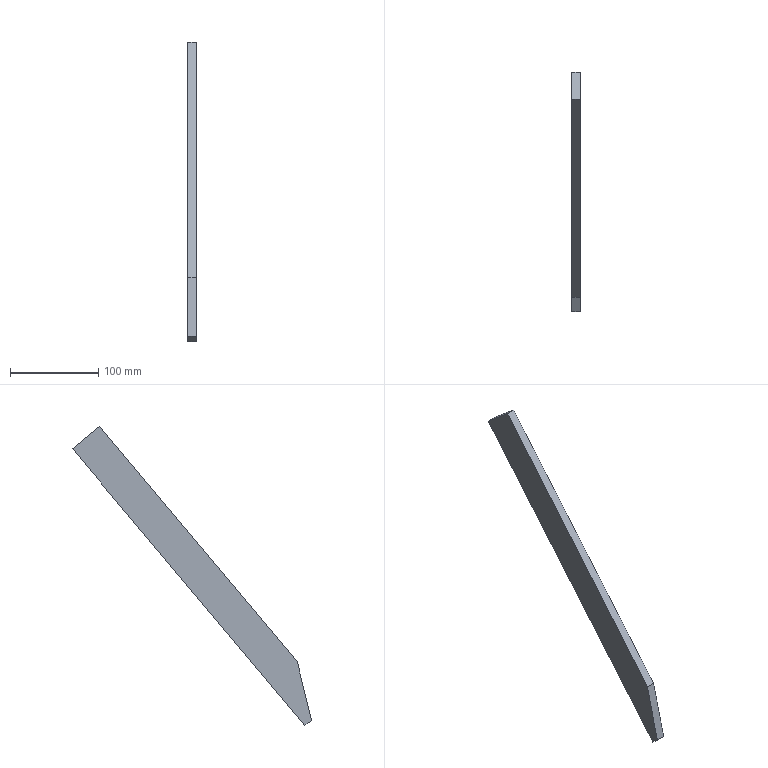Component | SolidWorks | Rebro sipke-1-100 | 1 solid | 7 faces | box 10 x 270.98 x 339.6 mm | volume 154755 mm3 | plane 7
build123d program:
from build123d import *

# Parameters (mm, degrees)
BOSS_EXTRUDE1_DEPTH = 10


with BuildPart() as part:
    # Sketch1 → Boss-Extrude1 (new body)
    with BuildSketch(Plane.XY):
        Polygon((0, 0), (0, 40), (409.712, 40), (409.712, 30), (348.847, 0), align=None)
    extrude(amount=BOSS_EXTRUDE1_DEPTH)


solid = part.part

# Placed as in the assembly
solid = solid.moved(Location((-1087.6, 322.096, -995.704), (-39.993, 90, 0)))
STEP:
#1=COLOUR_RGB('',0.7922,0.8196,0.9333);
#2=FILL_AREA_STYLE_COLOUR('',#1);
#3=FILL_AREA_STYLE('',(#2));
#4=SURFACE_STYLE_FILL_AREA(#3);
#5=SURFACE_SIDE_STYLE('',(#4));
#6=SURFACE_STYLE_USAGE(.BOTH.,#5);
#7=PRESENTATION_STYLE_ASSIGNMENT((#6));
#8=CARTESIAN_POINT('',(-42.819,12.681,-39.201));
#9=VERTEX_POINT('',#8);
#10=CARTESIAN_POINT('',(-42.819,3.854,-49.723));
#11=VERTEX_POINT('',#10);
#12=CARTESIAN_POINT('',(-42.819,12.681,-39.201));
#13=DIRECTION('',(0.,-0.6427,-0.7661));
#14=VECTOR('',#13,39.37);
#15=LINE('',#12,#14);
#16=EDGE_CURVE('',#9,#11,#15,.T.);
#17=ORIENTED_EDGE('',*,*,#16,.T.);
#18=CARTESIAN_POINT('',(-42.425,3.854,-49.723));
#19=VERTEX_POINT('',#18);
#20=CARTESIAN_POINT('',(-42.425,3.854,-49.723));
#21=DIRECTION('',(-1.,0.,-0.));
#22=VECTOR('',#21,39.37);
#23=LINE('',#20,#22);
#24=EDGE_CURVE('',#19,#11,#23,.T.);
#25=ORIENTED_EDGE('',*,*,#24,.F.);
#26=CARTESIAN_POINT('',(-42.425,12.681,-39.201));
#27=VERTEX_POINT('',#26);
#28=CARTESIAN_POINT('',(-42.425,12.681,-39.201));
#29=DIRECTION('',(0.,-0.6427,-0.7661));
#30=VECTOR('',#29,39.37);
#31=LINE('',#28,#30);
#32=EDGE_CURVE('',#27,#19,#31,.T.);
#33=ORIENTED_EDGE('',*,*,#32,.F.);
#34=CARTESIAN_POINT('',(-42.425,12.681,-39.201));
#35=DIRECTION('',(-1.,0.,-0.));
#36=VECTOR('',#35,39.37);
#37=LINE('',#34,#36);
#38=EDGE_CURVE('',#27,#9,#37,.T.);
#39=ORIENTED_EDGE('',*,*,#38,.T.);
#40=EDGE_LOOP('',(#17,#25,#33,#39));
#41=FACE_OUTER_BOUND('',#40,.T.);
#42=CARTESIAN_POINT('',(-42.425,12.681,-39.201));
#43=DIRECTION('',(0.,0.7661,-0.6427));
#44=DIRECTION('',(-0.,0.6427,0.7661));
#45=AXIS2_PLACEMENT_3D('',#42,#43,#44);
#46=PLANE('',#45);
#47=ADVANCED_FACE('',(#41),#46,.F.);
#48=CARTESIAN_POINT('',(-42.819,3.219,-52.318));
#49=VERTEX_POINT('',#48);
#50=CARTESIAN_POINT('',(-42.819,3.219,-52.318));
#51=DIRECTION('',(0.,-0.2378,-0.9713));
#52=VECTOR('',#51,39.37);
#53=LINE('',#50,#52);
#54=EDGE_CURVE('',#11,#49,#53,.T.);
#55=ORIENTED_EDGE('',*,*,#54,.T.);
#56=CARTESIAN_POINT('',(-42.425,3.219,-52.318));
#57=VERTEX_POINT('',#56);
#58=CARTESIAN_POINT('',(-42.425,3.219,-52.318));
#59=DIRECTION('',(-1.,0.,-0.));
#60=VECTOR('',#59,39.37);
#61=LINE('',#58,#60);
#62=EDGE_CURVE('',#57,#49,#61,.T.);
#63=ORIENTED_EDGE('',*,*,#62,.F.);
#64=CARTESIAN_POINT('',(-42.425,3.219,-52.318));
#65=DIRECTION('',(0.,-0.2378,-0.9713));
#66=VECTOR('',#65,39.37);
#67=LINE('',#64,#66);
#68=EDGE_CURVE('',#19,#57,#67,.T.);
#69=ORIENTED_EDGE('',*,*,#68,.F.);
#70=ORIENTED_EDGE('',*,*,#24,.T.);
#71=EDGE_LOOP('',(#55,#63,#69,#70));
#72=FACE_OUTER_BOUND('',#71,.T.);
#73=CARTESIAN_POINT('',(-42.425,3.219,-52.318));
#74=DIRECTION('',(0.,0.9713,-0.2378));
#75=DIRECTION('',(-0.,0.2378,0.9713));
#76=AXIS2_PLACEMENT_3D('',#73,#74,#75);
#77=PLANE('',#76);
#78=ADVANCED_FACE('',(#72),#77,.F.);
#79=CARTESIAN_POINT('',(-42.819,3.52,-52.571));
#80=VERTEX_POINT('',#79);
#81=CARTESIAN_POINT('',(-42.819,3.219,-52.318));
#82=DIRECTION('',(0.,0.7661,-0.6427));
#83=VECTOR('',#82,39.37);
#84=LINE('',#81,#83);
#85=EDGE_CURVE('',#49,#80,#84,.T.);
#86=ORIENTED_EDGE('',*,*,#85,.T.);
#87=CARTESIAN_POINT('',(-42.425,3.52,-52.571));
#88=VERTEX_POINT('',#87);
#89=CARTESIAN_POINT('',(-42.425,3.52,-52.571));
#90=DIRECTION('',(-1.,0.,-0.));
#91=VECTOR('',#90,39.37);
#92=LINE('',#89,#91);
#93=EDGE_CURVE('',#88,#80,#92,.T.);
#94=ORIENTED_EDGE('',*,*,#93,.F.);
#95=CARTESIAN_POINT('',(-42.425,3.219,-52.318));
#96=DIRECTION('',(0.,0.7661,-0.6427));
#97=VECTOR('',#96,39.37);
#98=LINE('',#95,#97);
#99=EDGE_CURVE('',#57,#88,#98,.T.);
#100=ORIENTED_EDGE('',*,*,#99,.F.);
#101=ORIENTED_EDGE('',*,*,#62,.T.);
#102=EDGE_LOOP('',(#86,#94,#100,#101));
#103=FACE_OUTER_BOUND('',#102,.T.);
#104=CARTESIAN_POINT('',(-42.425,3.219,-52.318));
#105=DIRECTION('',(-0.,0.6427,0.7661));
#106=DIRECTION('',(1.,-0.,0.));
#107=AXIS2_PLACEMENT_3D('',#104,#105,#106);
#108=PLANE('',#107);
#109=ADVANCED_FACE('',(#103),#108,.F.);
#110=CARTESIAN_POINT('',(-42.819,13.887,-40.213));
#111=VERTEX_POINT('',#110);
#112=CARTESIAN_POINT('',(-42.819,13.887,-40.213));
#113=DIRECTION('',(-0.,0.6427,0.7661));
#114=VECTOR('',#113,39.37);
#115=LINE('',#112,#114);
#116=EDGE_CURVE('',#80,#111,#115,.T.);
#117=ORIENTED_EDGE('',*,*,#116,.T.);
#118=CARTESIAN_POINT('',(-42.425,13.887,-40.213));
#119=VERTEX_POINT('',#118);
#120=CARTESIAN_POINT('',(-42.425,13.887,-40.213));
#121=DIRECTION('',(-1.,0.,-0.));
#122=VECTOR('',#121,39.37);
#123=LINE('',#120,#122);
#124=EDGE_CURVE('',#119,#111,#123,.T.);
#125=ORIENTED_EDGE('',*,*,#124,.F.);
#126=CARTESIAN_POINT('',(-42.425,13.887,-40.213));
#127=DIRECTION('',(-0.,0.6427,0.7661));
#128=VECTOR('',#127,39.37);
#129=LINE('',#126,#128);
#130=EDGE_CURVE('',#88,#119,#129,.T.);
#131=ORIENTED_EDGE('',*,*,#130,.F.);
#132=ORIENTED_EDGE('',*,*,#93,.T.);
#133=EDGE_LOOP('',(#117,#125,#131,#132));
#134=FACE_OUTER_BOUND('',#133,.T.);
#135=CARTESIAN_POINT('',(-42.425,13.887,-40.213));
#136=DIRECTION('',(-0.,-0.7661,0.6427));
#137=DIRECTION('',(0.,-0.6427,-0.7661));
#138=AXIS2_PLACEMENT_3D('',#135,#136,#137);
#139=PLANE('',#138);
#140=ADVANCED_FACE('',(#134),#139,.F.);
#141=CARTESIAN_POINT('',(-42.819,12.681,-39.201));
#142=DIRECTION('',(-0.,-0.7661,0.6427));
#143=VECTOR('',#142,39.37);
#144=LINE('',#141,#143);
#145=EDGE_CURVE('',#111,#9,#144,.T.);
#146=ORIENTED_EDGE('',*,*,#145,.T.);
#147=ORIENTED_EDGE('',*,*,#38,.F.);
#148=CARTESIAN_POINT('',(-42.425,12.681,-39.201));
#149=DIRECTION('',(-0.,-0.7661,0.6427));
#150=VECTOR('',#149,39.37);
#151=LINE('',#148,#150);
#152=EDGE_CURVE('',#119,#27,#151,.T.);
#153=ORIENTED_EDGE('',*,*,#152,.F.);
#154=ORIENTED_EDGE('',*,*,#124,.T.);
#155=EDGE_LOOP('',(#146,#147,#153,#154));
#156=FACE_OUTER_BOUND('',#155,.T.);
#157=CARTESIAN_POINT('',(-42.425,12.681,-39.201));
#158=DIRECTION('',(0.,-0.6427,-0.7661));
#159=DIRECTION('',(0.,0.7661,-0.6427));
#160=AXIS2_PLACEMENT_3D('',#157,#158,#159);
#161=PLANE('',#160);
#162=ADVANCED_FACE('',(#156),#161,.F.);
#163=ORIENTED_EDGE('',*,*,#32,.T.);
#164=ORIENTED_EDGE('',*,*,#68,.T.);
#165=ORIENTED_EDGE('',*,*,#99,.T.);
#166=ORIENTED_EDGE('',*,*,#130,.T.);
#167=ORIENTED_EDGE('',*,*,#152,.T.);
#168=EDGE_LOOP('',(#163,#164,#165,#166,#167));
#169=FACE_OUTER_BOUND('',#168,.T.);
#170=CARTESIAN_POINT('',(-42.425,12.681,-39.201));
#171=DIRECTION('',(1.,-0.,0.));
#172=DIRECTION('',(0.,-0.6427,-0.7661));
#173=AXIS2_PLACEMENT_3D('',#170,#171,#172);
#174=PLANE('',#173);
#175=ADVANCED_FACE('',(#169),#174,.T.);
#176=ORIENTED_EDGE('',*,*,#16,.F.);
#177=ORIENTED_EDGE('',*,*,#145,.F.);
#178=ORIENTED_EDGE('',*,*,#116,.F.);
#179=ORIENTED_EDGE('',*,*,#85,.F.);
#180=ORIENTED_EDGE('',*,*,#54,.F.);
#181=EDGE_LOOP('',(#176,#177,#178,#179,#180));
#182=FACE_OUTER_BOUND('',#181,.T.);
#183=CARTESIAN_POINT('',(-42.819,12.681,-39.201));
#184=DIRECTION('',(1.,-0.,0.));
#185=DIRECTION('',(0.,-0.6427,-0.7661));
#186=AXIS2_PLACEMENT_3D('',#183,#184,#185);
#187=PLANE('',#186);
#188=ADVANCED_FACE('',(#182),#187,.F.);
#189=CLOSED_SHELL('',(#47,#78,#109,#140,#162,#175,#188));
#190=MANIFOLD_SOLID_BREP('',#189);
#191=STYLED_ITEM('',(#7),#190);
#192=PRESENTATION_LAYER_ASSIGNMENT('','',(#191));
#193=CARTESIAN_POINT('',(0.,0.,0.));
#194=DIRECTION('',(0.,0.,1.));
#195=DIRECTION('',(1.,0.,0.));
#196=AXIS2_PLACEMENT_3D('',#193,#194,#195);
#197=(LENGTH_UNIT()NAMED_UNIT(*)SI_UNIT($,.METRE.));
#198=LENGTH_MEASURE_WITH_UNIT(LENGTH_MEASURE(0.0254),#197);
#199=DIMENSIONAL_EXPONENTS(1.,0.,0.,0.,0.,0.,0.);
#200=(CONVERSION_BASED_UNIT('',#198)LENGTH_UNIT()NAMED_UNIT(#199));
#201=UNCERTAINTY_MEASURE_WITH_UNIT(LENGTH_MEASURE(0.00001),#200,'','');
#202=(NAMED_UNIT(*)PLANE_ANGLE_UNIT()SI_UNIT($,.RADIAN.));
#203=(NAMED_UNIT(*)SI_UNIT($,.STERADIAN.)SOLID_ANGLE_UNIT());
#204=(GEOMETRIC_REPRESENTATION_CONTEXT(3)GLOBAL_UNCERTAINTY_ASSIGNED_CONTEXT((#201))GLOBAL_UNIT_ASSIGNED_CONTEXT((#200,#202,#203))REPRESENTATION_CONTEXT('',''));
#205=ADVANCED_BREP_SHAPE_REPRESENTATION('',(#190,#196),#204);
#206=(LENGTH_UNIT()NAMED_UNIT(*)SI_UNIT($,.METRE.));
#207=LENGTH_MEASURE_WITH_UNIT(LENGTH_MEASURE(0.0254),#206);
#208=DIMENSIONAL_EXPONENTS(1.,0.,0.,0.,0.,0.,0.);
#209=(CONVERSION_BASED_UNIT('',#207)LENGTH_UNIT()NAMED_UNIT(#208));
#210=UNCERTAINTY_MEASURE_WITH_UNIT(LENGTH_MEASURE(0.00001),#209,'','');
#211=(NAMED_UNIT(*)PLANE_ANGLE_UNIT()SI_UNIT($,.RADIAN.));
#212=(NAMED_UNIT(*)SI_UNIT($,.STERADIAN.)SOLID_ANGLE_UNIT());
#213=(GEOMETRIC_REPRESENTATION_CONTEXT(3)GLOBAL_UNCERTAINTY_ASSIGNED_CONTEXT((#210))GLOBAL_UNIT_ASSIGNED_CONTEXT((#209,#211,#212))REPRESENTATION_CONTEXT('',''));
#214=MECHANICAL_DESIGN_GEOMETRIC_PRESENTATION_REPRESENTATION('',(#191),#213);